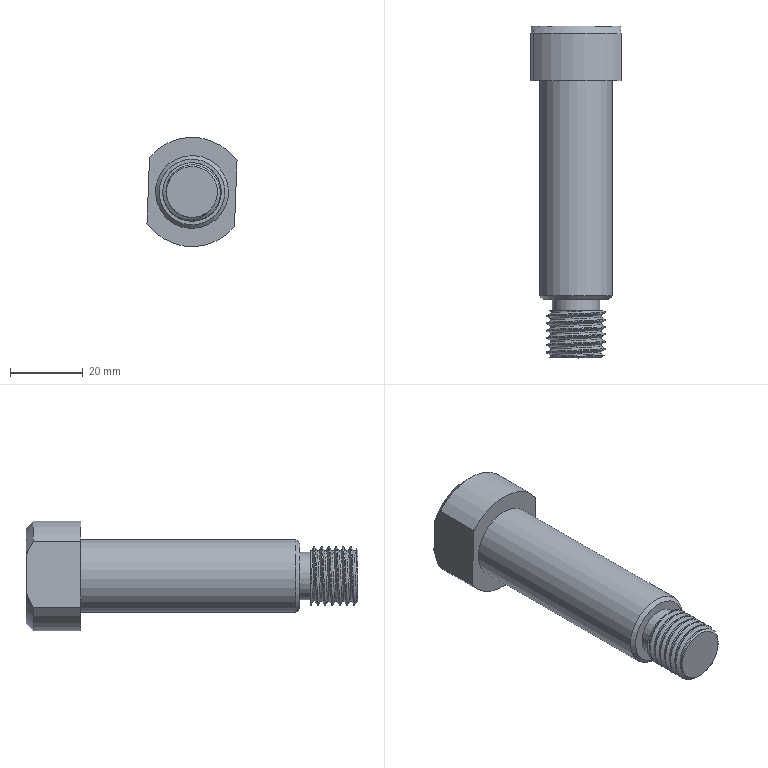Component | NX | SHORT_PIN_2 | 1 solid | 19 faces | volume 30860 mm3 | plane 7 | cylinder 6 | cone 4 | spline 2 | commonest cylinder face diameters 30 x2 20 x1 13 x1 16 x1 14 x1